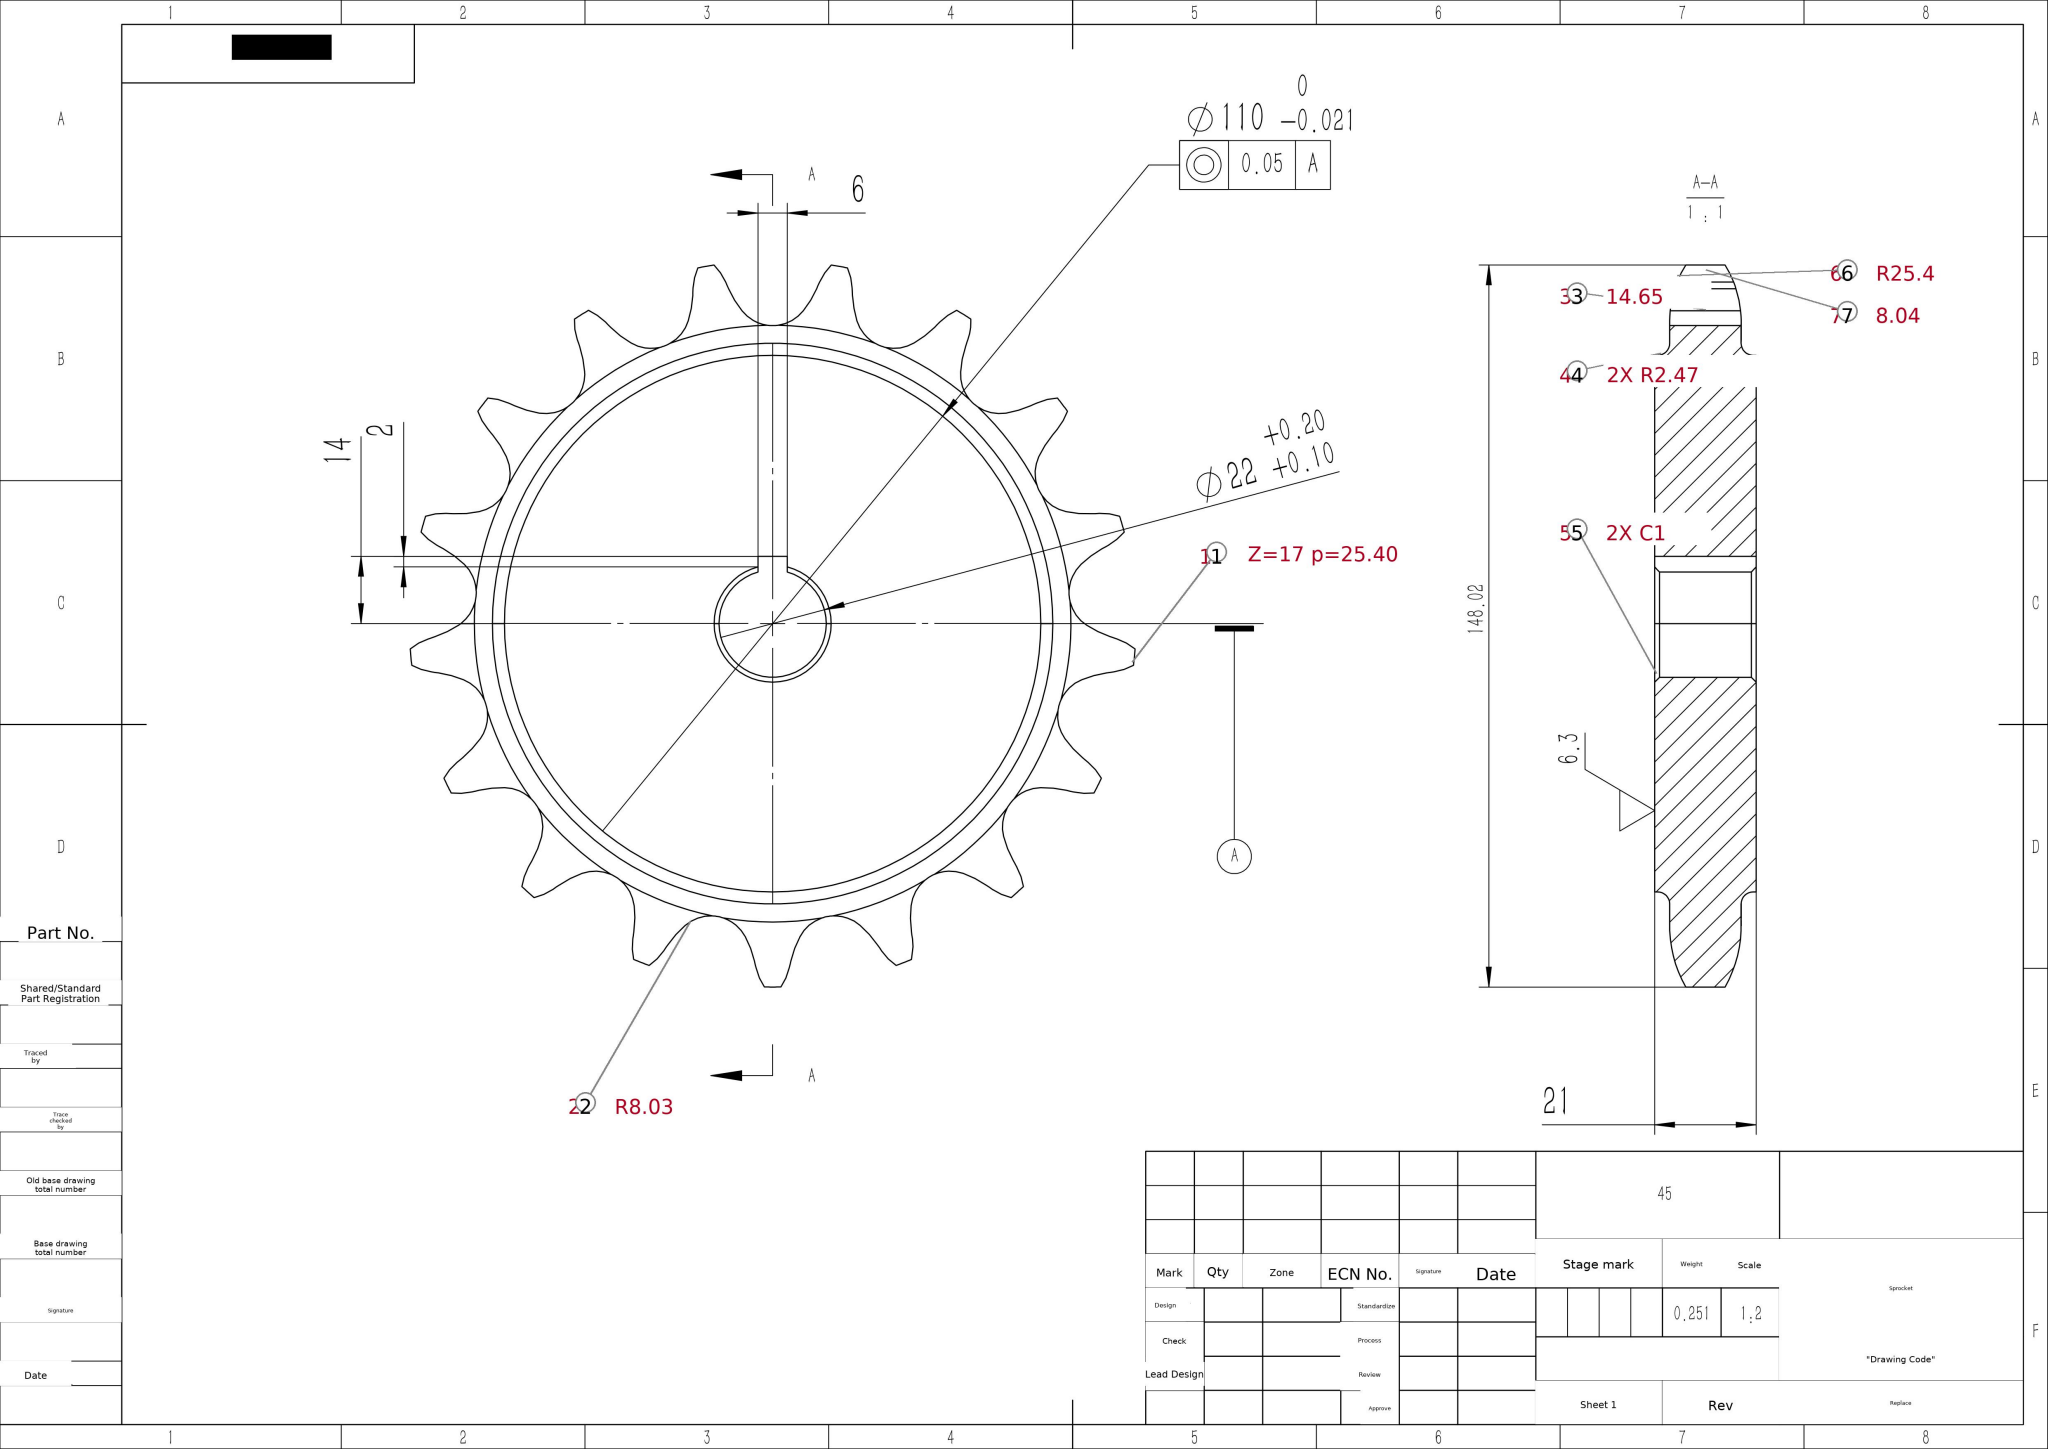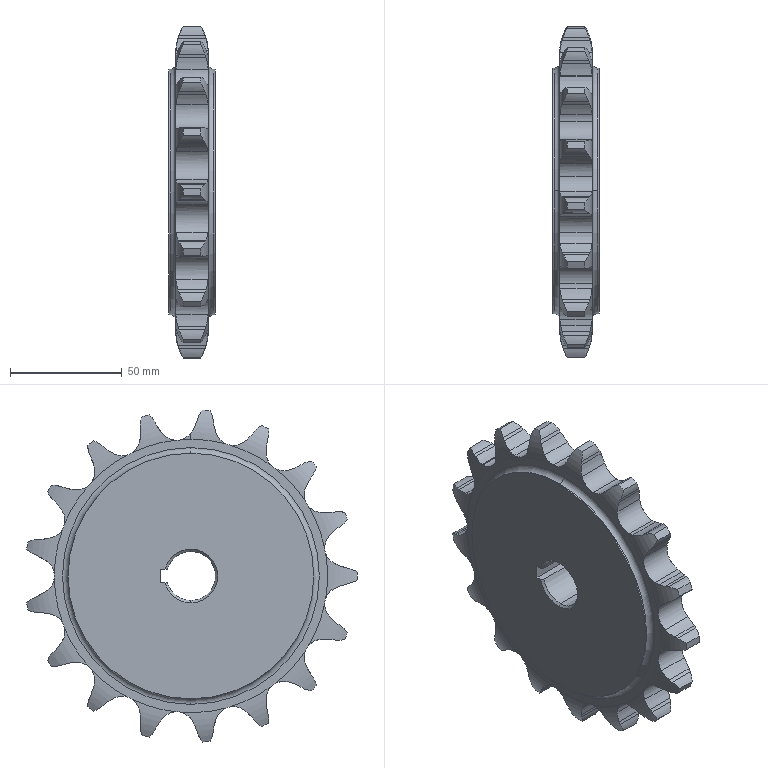Part | SolidWorks | mm | 1 solid | 204 faces | box 20.82 x 148.02 x 148.64 mm | volume 250839 mm3 | cylinder 117 | plane 41 | torus 40 | cone 6 | commonest cylinder face diameters 23.3 x36 41.467 x35 16.059 x22 149 x17 110 x4 22 x3